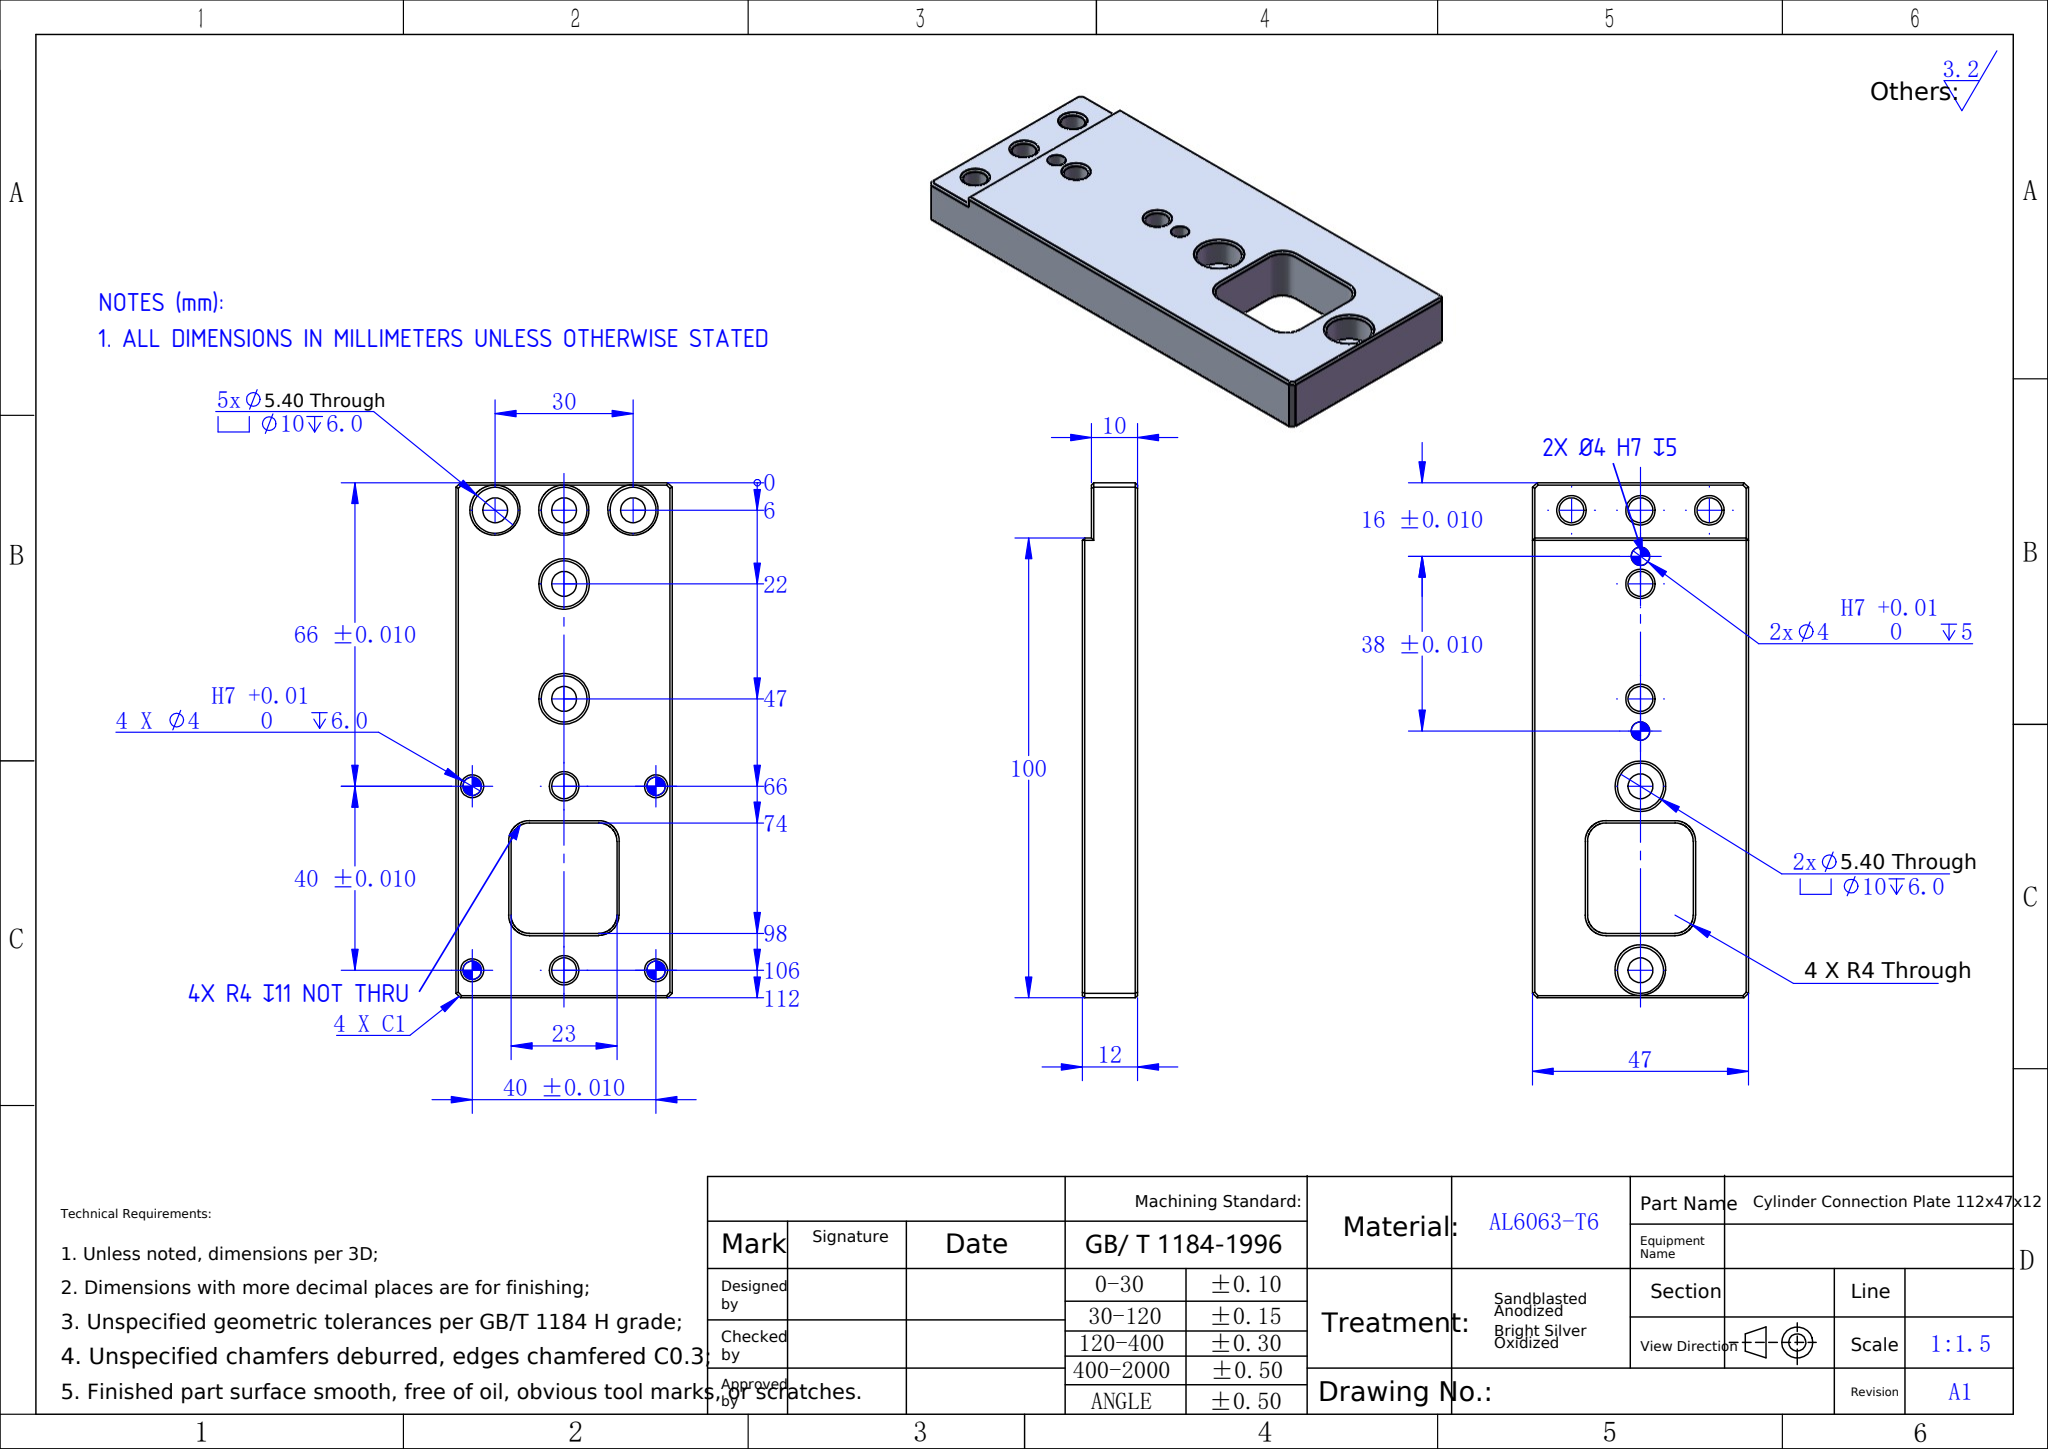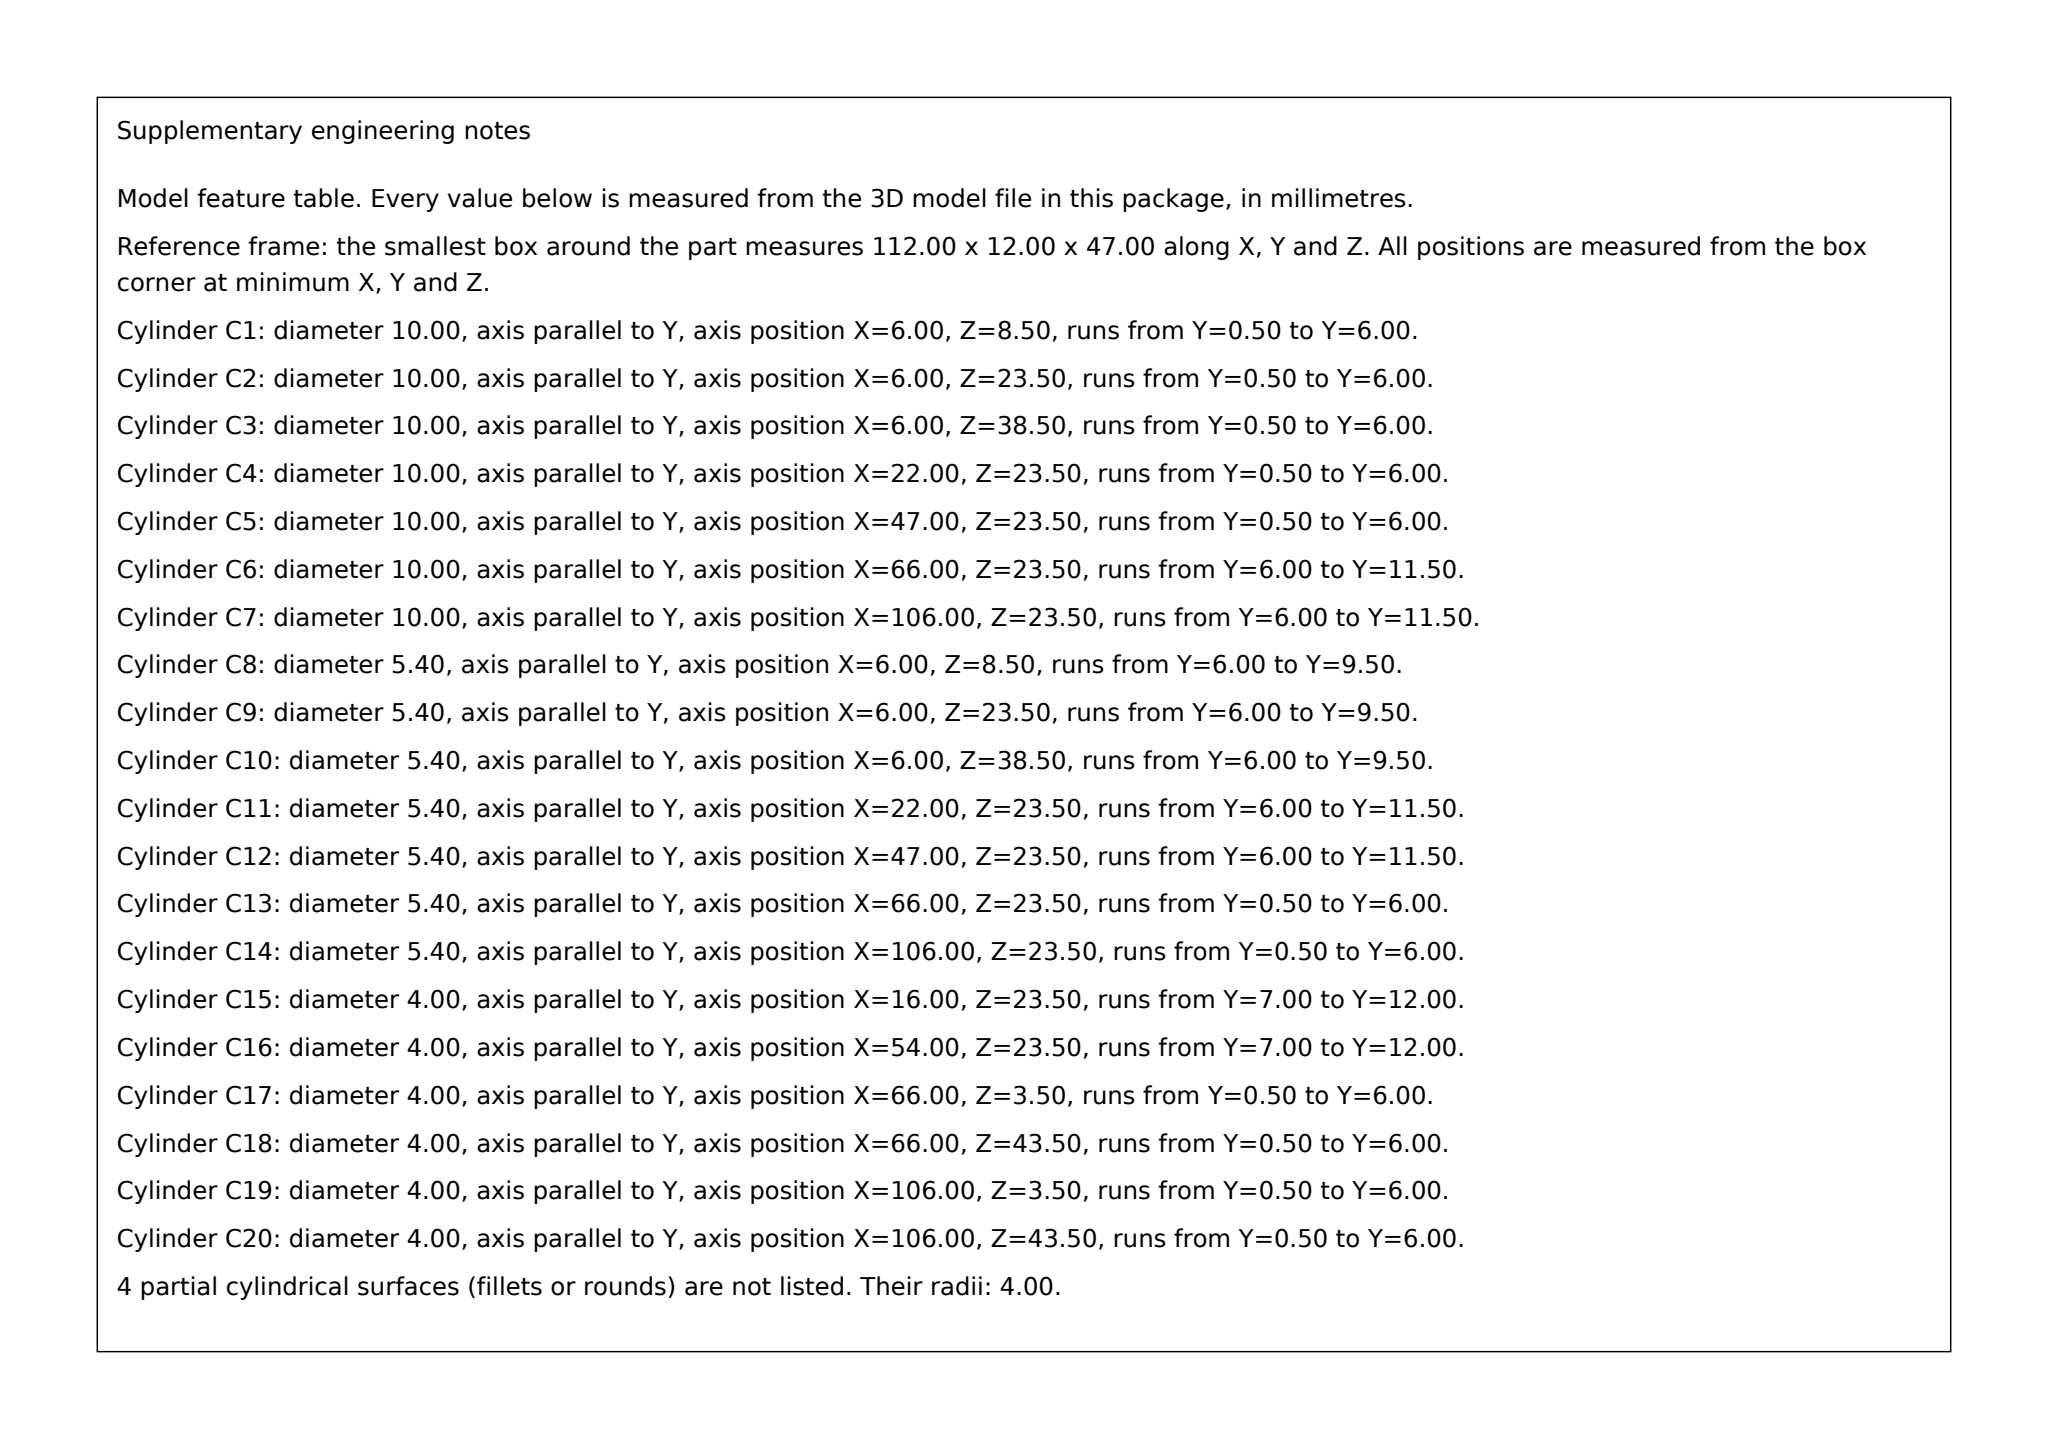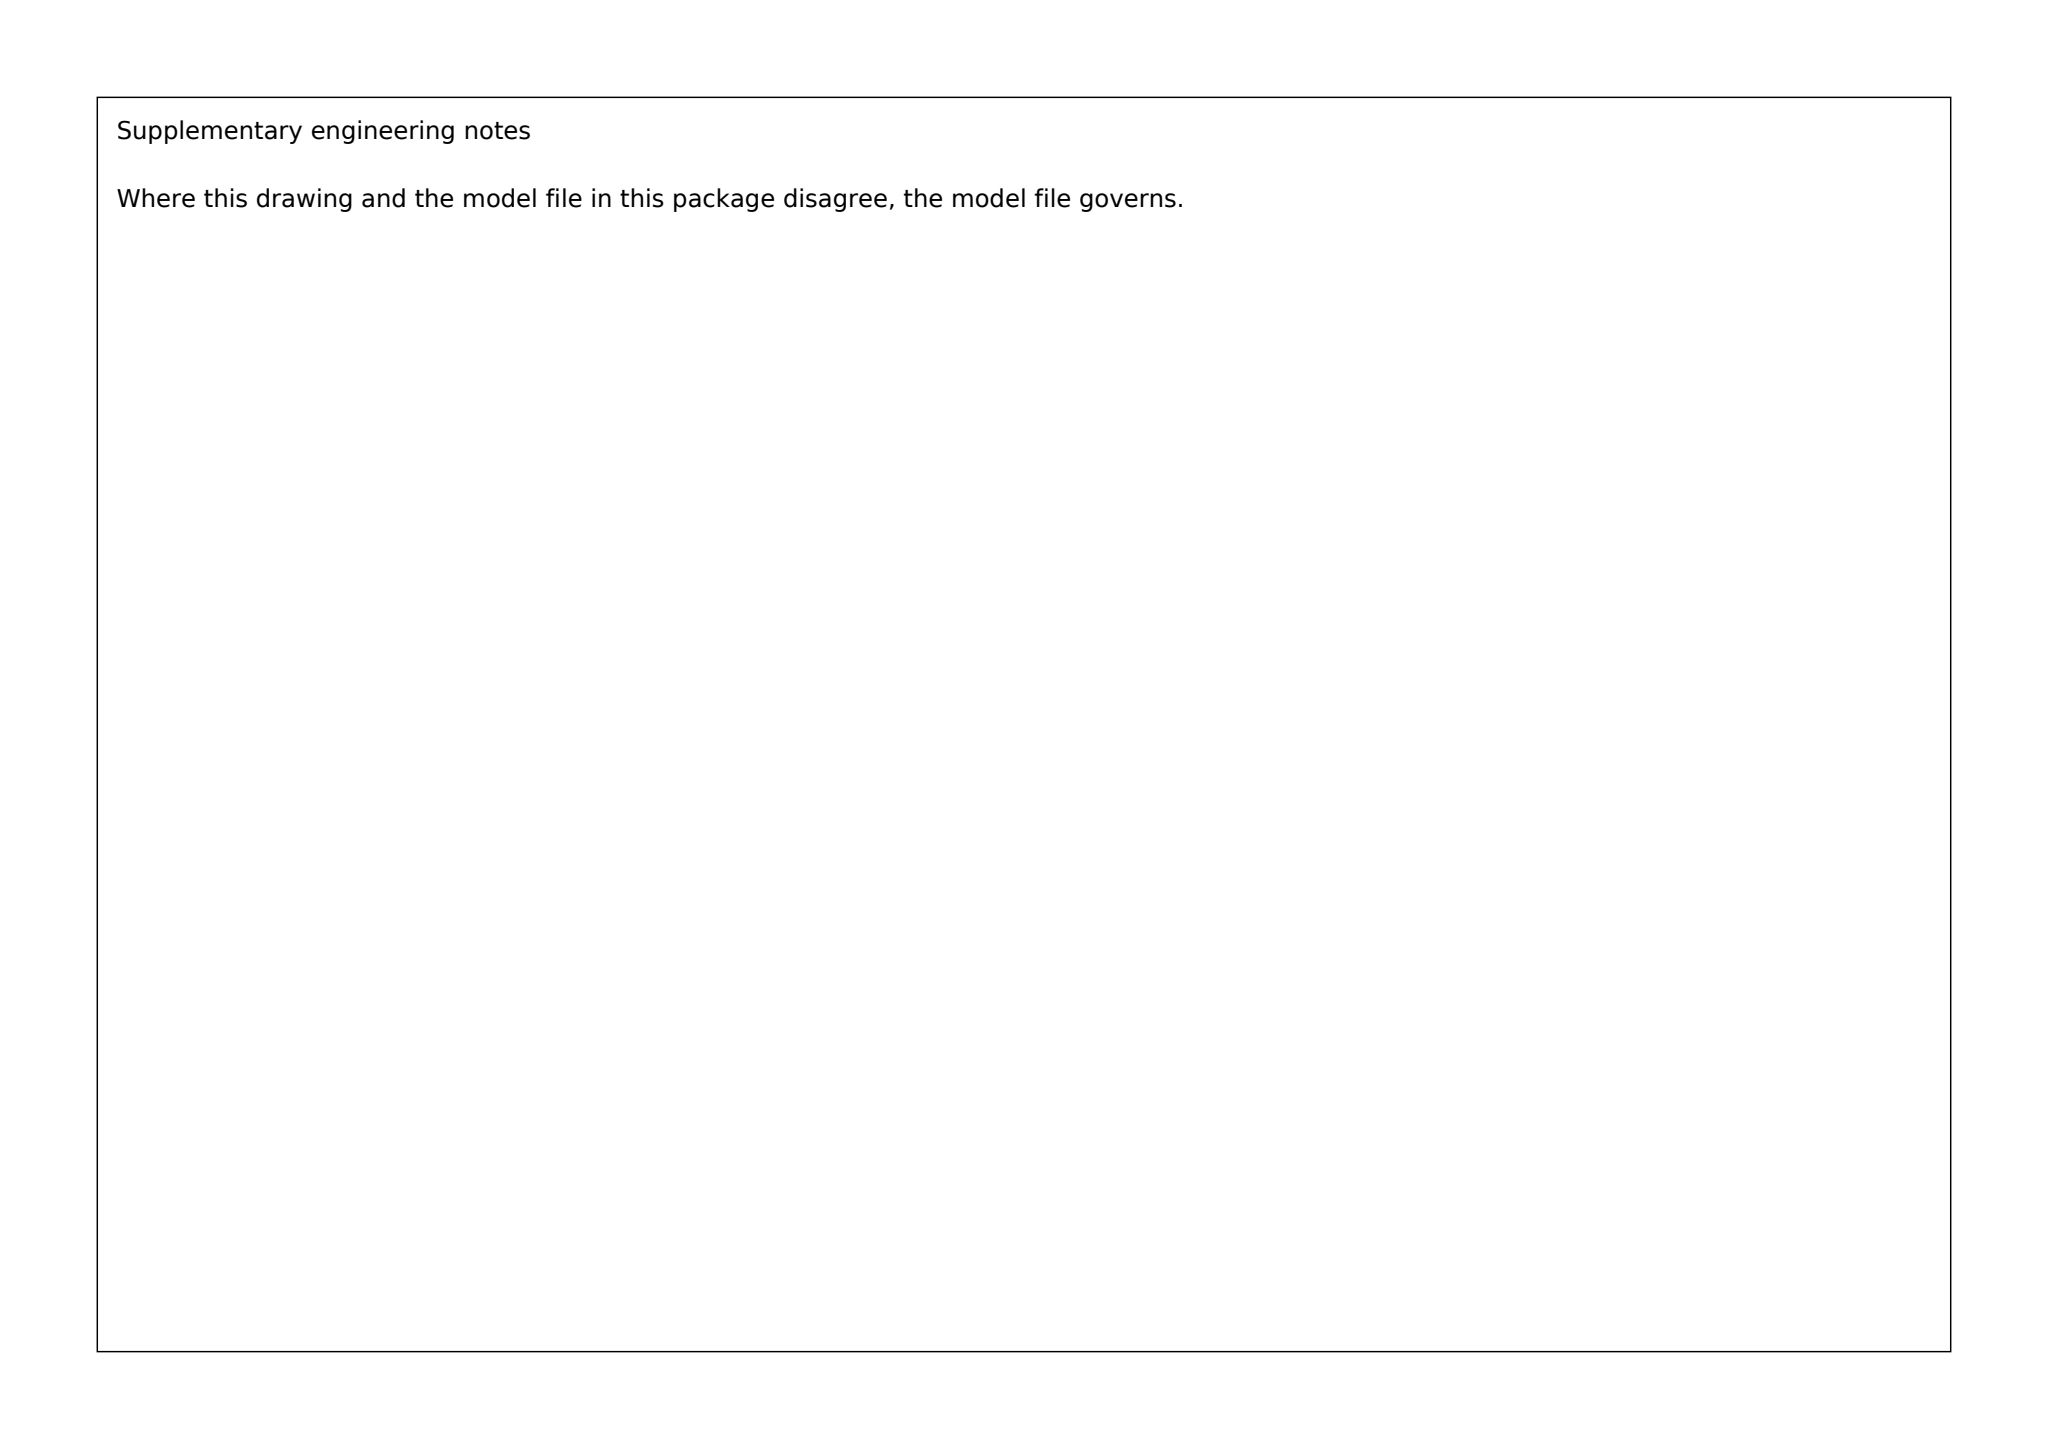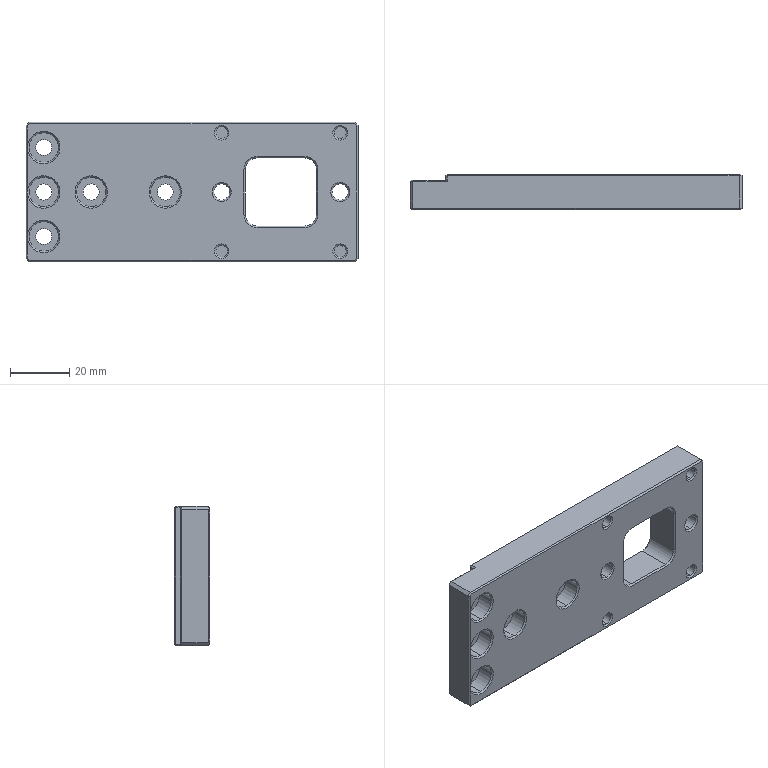Part | SolidWorks | mm | material AL6063-T6 | 1 solid | 148 faces | box 112 x 12 x 47 mm | volume 50850 mm3 | plane 60 | cylinder 44 | cone 44 | commonest cylinder face diameters 10 x14 5.4 x14 4 x12 8 x4
Drawing notes:
ALL DIMENSIONS IN MILLIMETERS UNLESS OTHERWISE STATED | from the solid: STEP bbox_xyz = 112.0 x 12.0 x 47.0 mm (model units mm)
2X Ø4 H7 ⍌5 (SIDE VIEW) NOT SAME AS 4X Ø4 H7 ⍌6.0 (FRONT) | from the solid: Ø4 cyls len 5.0 at x=16 & 54, z=23.5; separate Ø4 len 5.5+C at x=66,106, z=3.5/43.5
4X R4 PKT CNRS: ⍌11 FROM TOP FACE, NOT THRU | from the solid: Ø8 cyls len 11.0 at (78,16),(78,31),(94,16),(94,31); part 12 thick